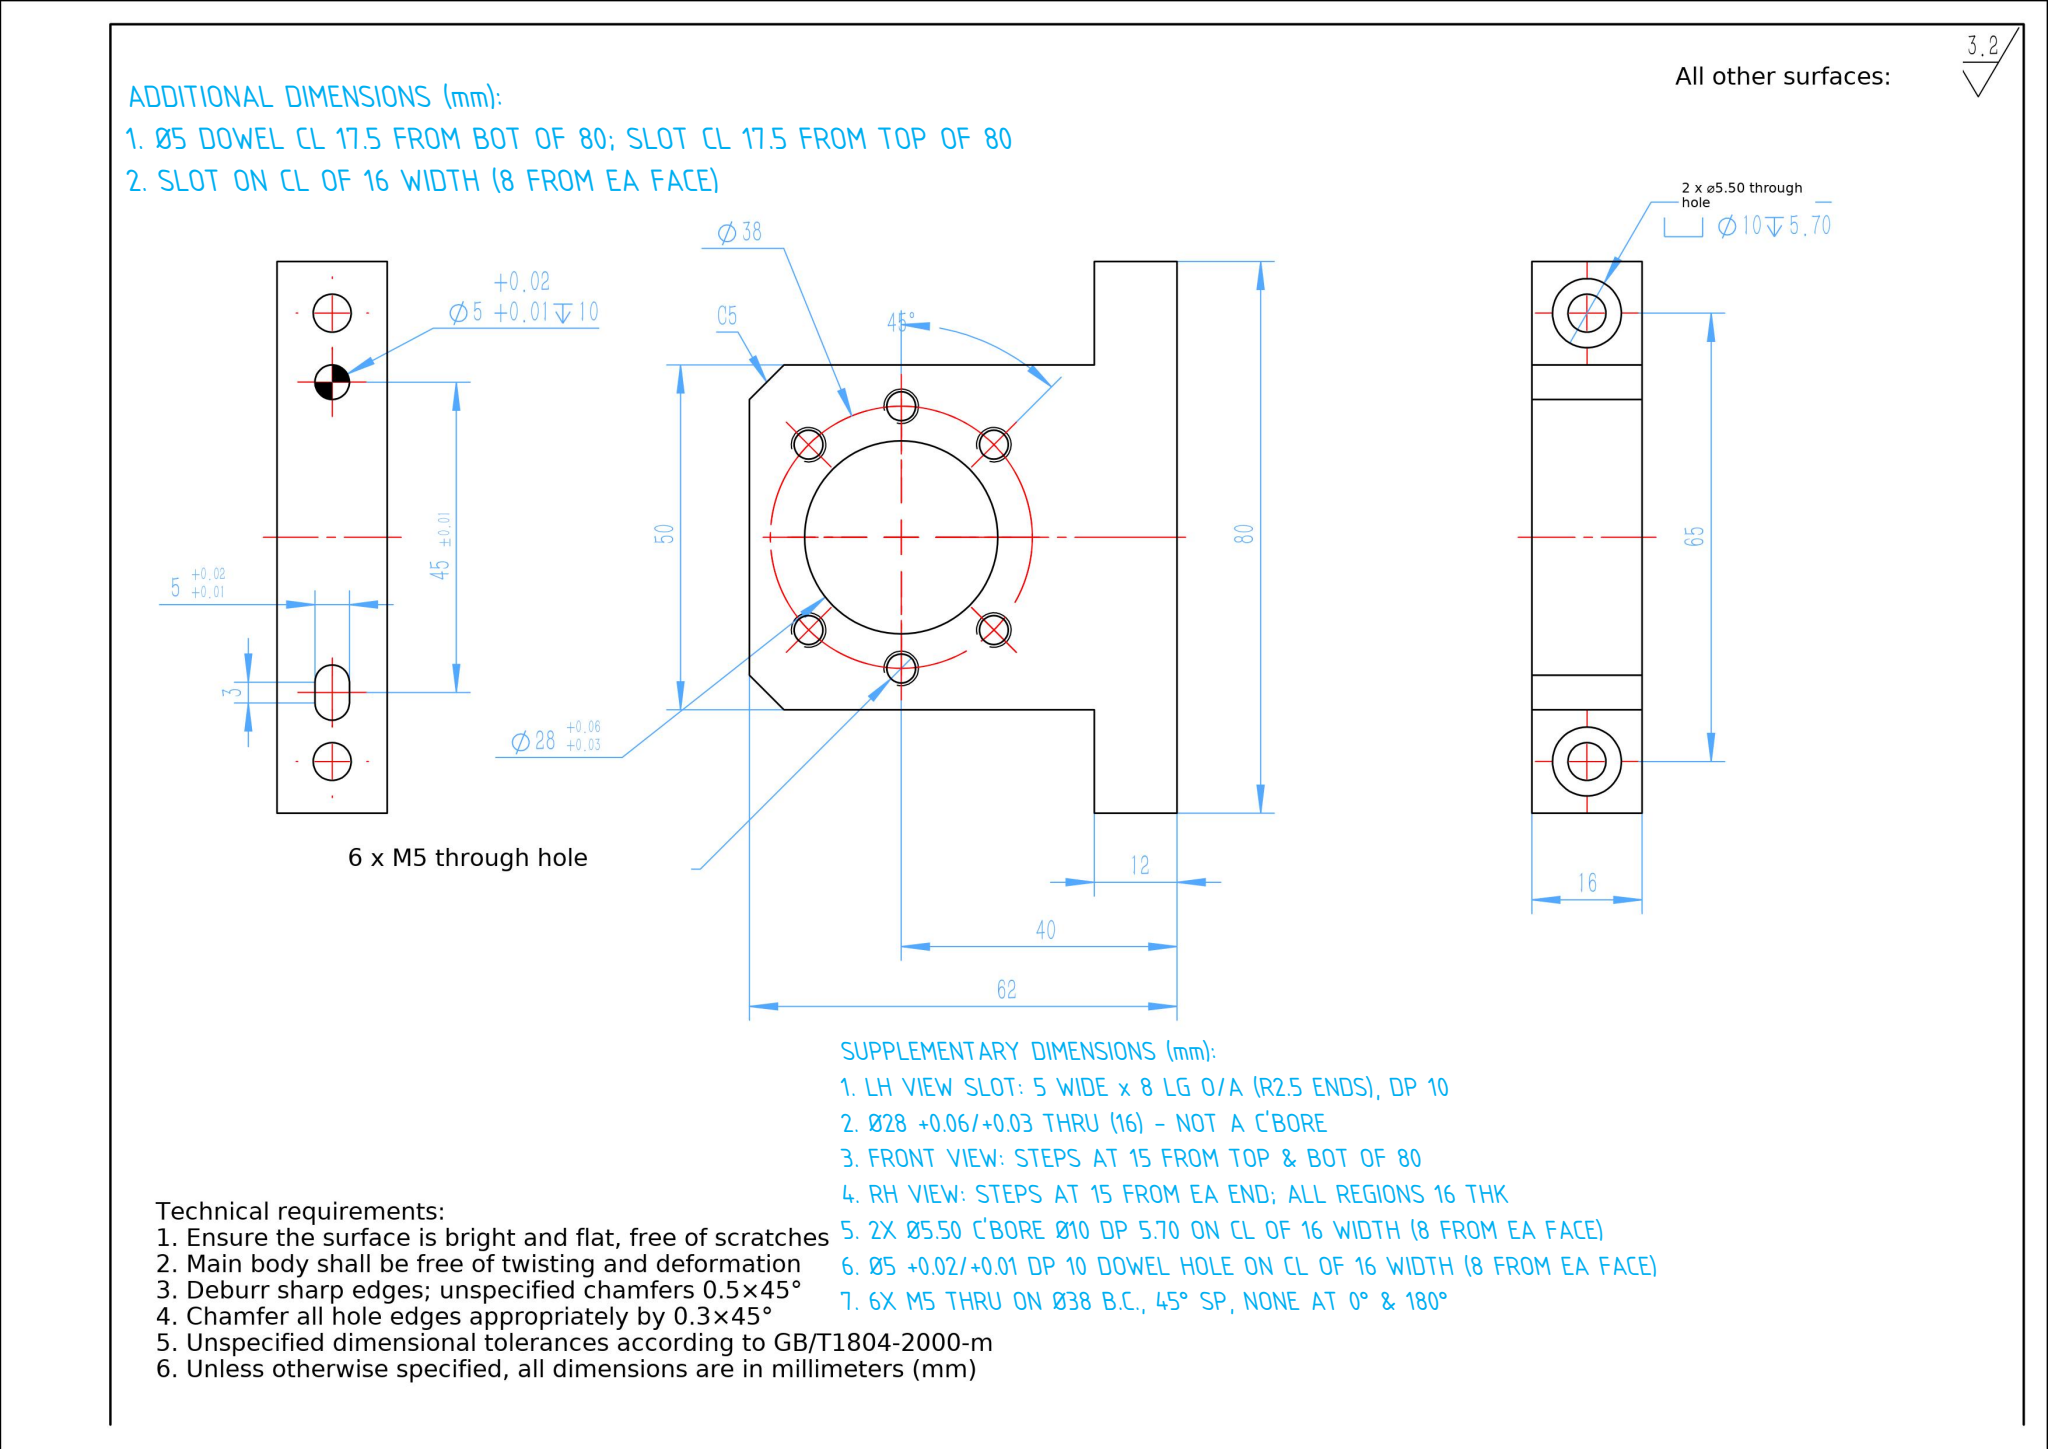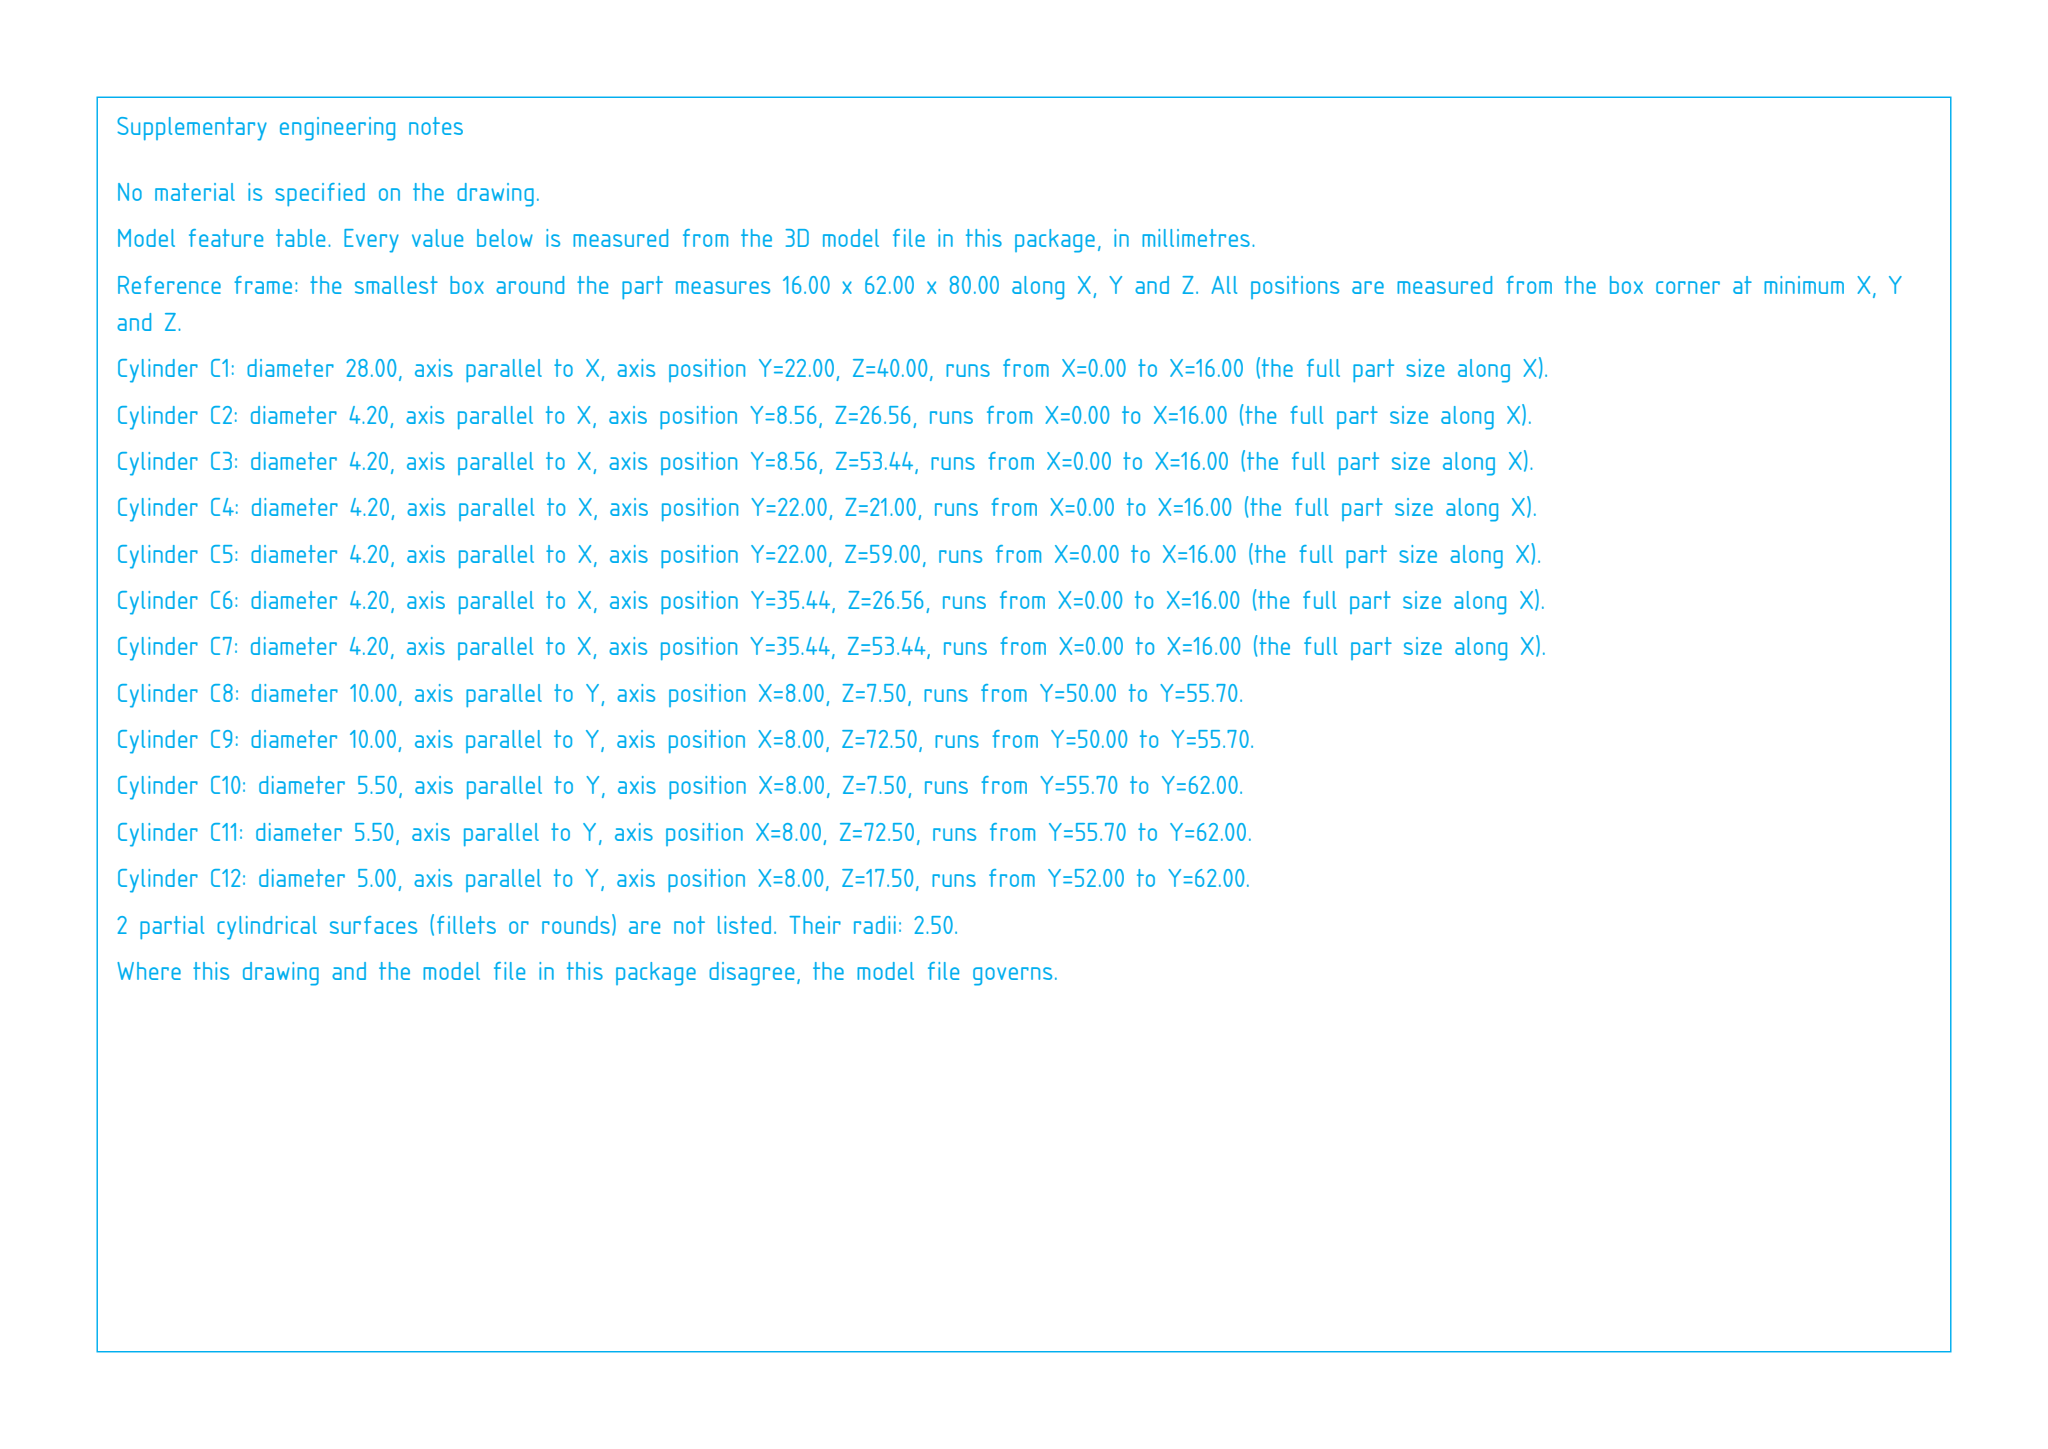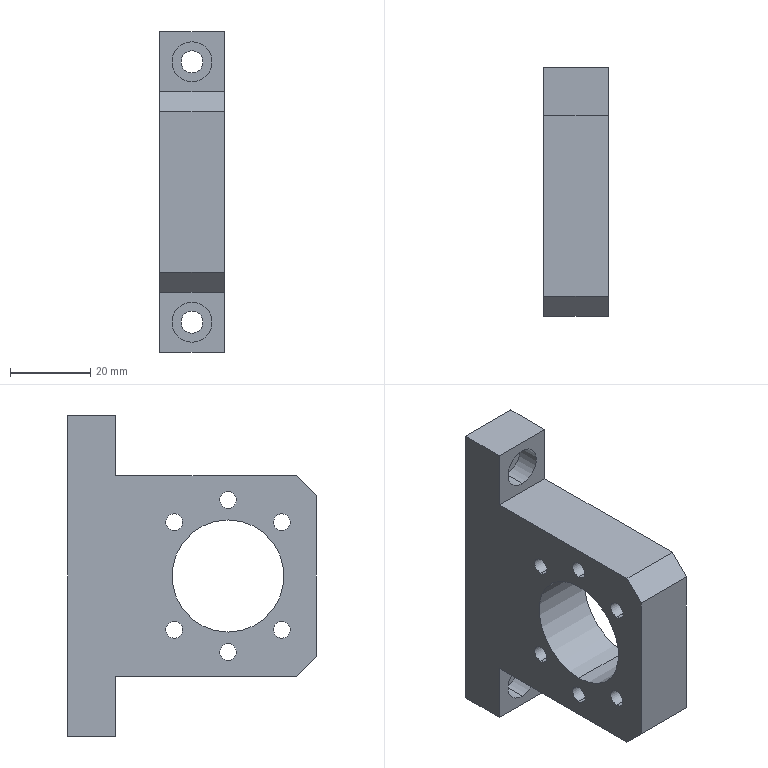Part | SolidWorks | mm | 1 solid | 45 faces | box 16 x 62 x 80 mm | volume 42041 mm3 | cylinder 27 | plane 18 | commonest cylinder face diameters 4.2 x12 5 x5 10 x4 5.5 x4 28 x2
build123d program:
from build123d import *

# Parameters (mm, degrees)
BOSS_EXTRUDE1_DEPTH                               = 8
SKETCH2_R                                         = 14
CUT_EXTRUDE1_DEPTH                                = 76.498
CHAMFER1_SIZE                                     = 5
HOLE_SIZE_ACCORDING_TO_TYPE_1_OF_HEXA_D           = 5.5
HOLE_SIZE_ACCORDING_TO_TYPE_1_OF_HEXA_CBORE_D     = 10
HOLE_SIZE_ACCORDING_TO_TYPE_1_OF_HEXA_CBORE_DEPTH = 5.7
M5_TAPPED_HOLE1_D                                 = 4.2
SKETCH7_R                                         = 2.5
CUT_EXTRUDE2_DEPTH                                = 10


with BuildPart() as part:
    # Sketch1 → Boss-Extrude1 (new, symmetric)
    with BuildSketch(Plane(origin=(0, 0, 0), x_dir=(0, 0, -1), z_dir=(1, 0, 0))):
        Polygon((-40, 0), (40, 0), (40, -12), (25, -12), (25, -62), (-25, -62), (-25, -12), (-40, -12), align=None)
    extrude(amount=BOSS_EXTRUDE1_DEPTH, both=True)

    # Sketch2 → Cut-Extrude1 (cut, through all)
    with BuildSketch(Plane(origin=(8, 0, 0), x_dir=(0, 0, -1), z_dir=(1, 0, 0))):
        with Locations((0, -40)):
            Circle(SKETCH2_R)
    extrude(amount=-CUT_EXTRUDE1_DEPTH, mode=Mode.SUBTRACT)

    # Chamfer1
    chamfer1_edges = [part.edges().sort_by_distance(p)[0] for p in [
        (0, -62, -25),
        (0, -62, 25),
    ]]
    chamfer(chamfer1_edges, length=CHAMFER1_SIZE)

    # Hole Size _ according to_ Type 1 of Hexa (through all)
    with Locations(Plane(origin=(0, -12, 0), x_dir=(-1, 0, 0), z_dir=(0, -1, 0))):
        with Locations((0, -32.5), (0, 32.5)):
            CounterBoreHole(HOLE_SIZE_ACCORDING_TO_TYPE_1_OF_HEXA_D / 2, HOLE_SIZE_ACCORDING_TO_TYPE_1_OF_HEXA_CBORE_D / 2, HOLE_SIZE_ACCORDING_TO_TYPE_1_OF_HEXA_CBORE_DEPTH)

    # M5 Tapped Hole1 (through all)
    with Locations(Plane(origin=(8, 0, 0), x_dir=(0, 0, -1), z_dir=(1, 0, 0))):
        with Locations((-13.435, -26.565), (-19, -40), (19, -40), (13.435, -26.565), (-13.435, -53.435), (13.435, -53.435)):
            Hole(M5_TAPPED_HOLE1_D / 2)

    # Sketch7 → Cut-Extrude2 (cut)
    with BuildSketch(Plane(origin=(0, 0, 0), x_dir=(1, 0, 0), z_dir=(0, 1, 0))):
        with Locations(Location((0, 22.5, 0), (0, 0, 270))):
            Circle(SKETCH7_R)
        with BuildLine():
            Line((-2.5, -24), (-2.5, -21))
            ThreePointArc((-2.5, -21), (0, -18.5), (2.5, -21))
            Line((2.5, -21), (2.5, -24))
            ThreePointArc((2.5, -24), (0, -26.5), (-2.5, -24))
        make_face()
    extrude(amount=-CUT_EXTRUDE2_DEPTH, mode=Mode.SUBTRACT)


solid = part.part